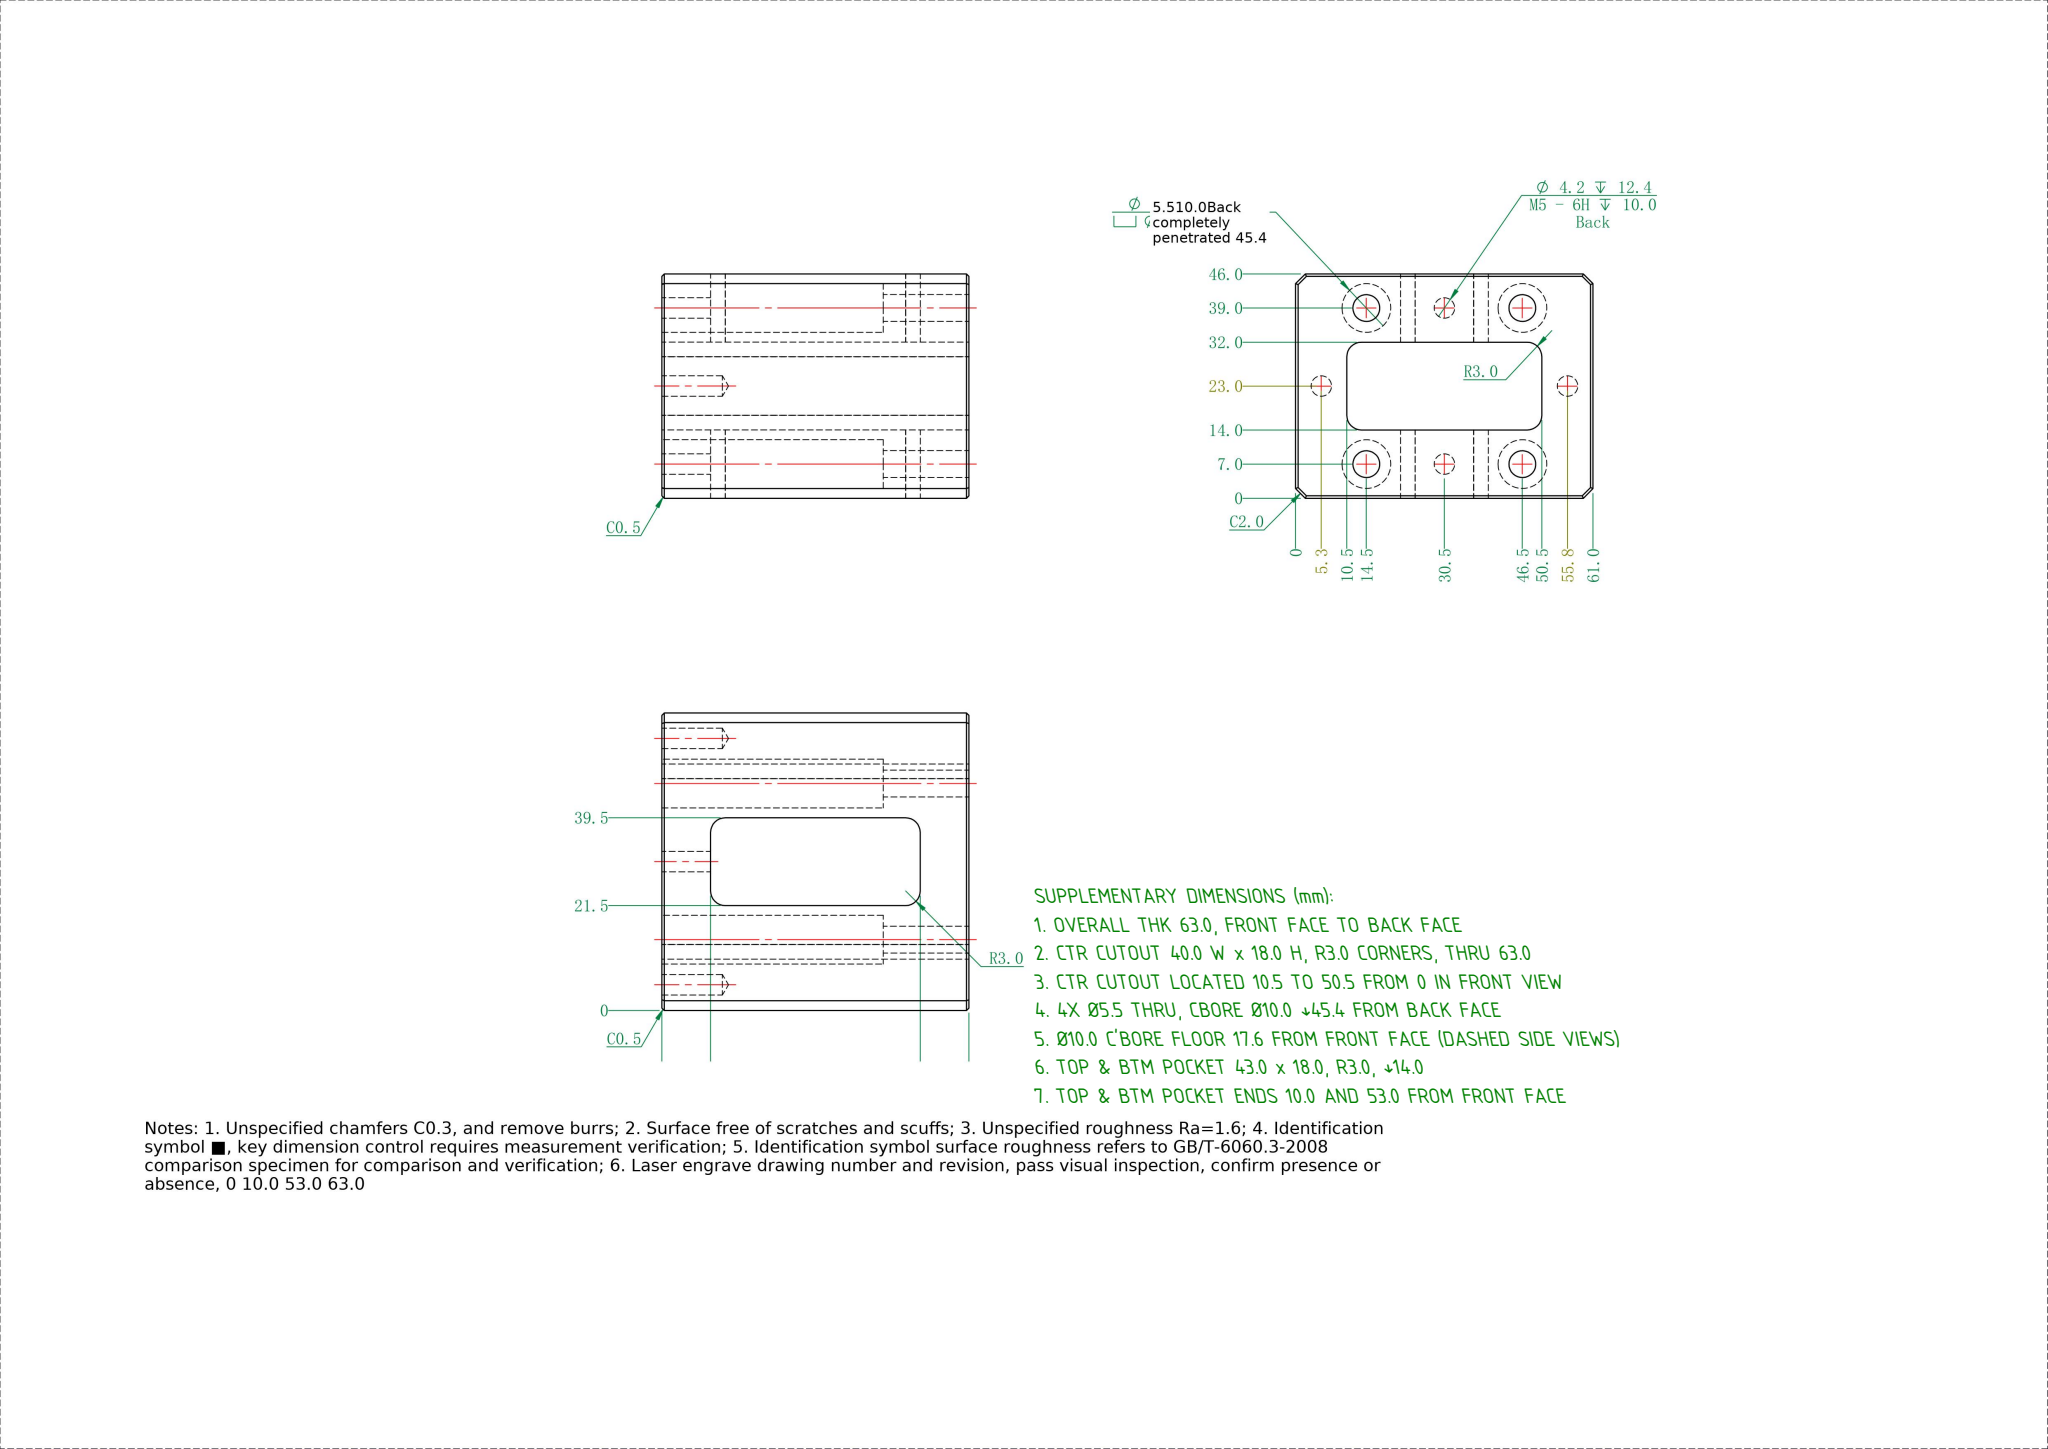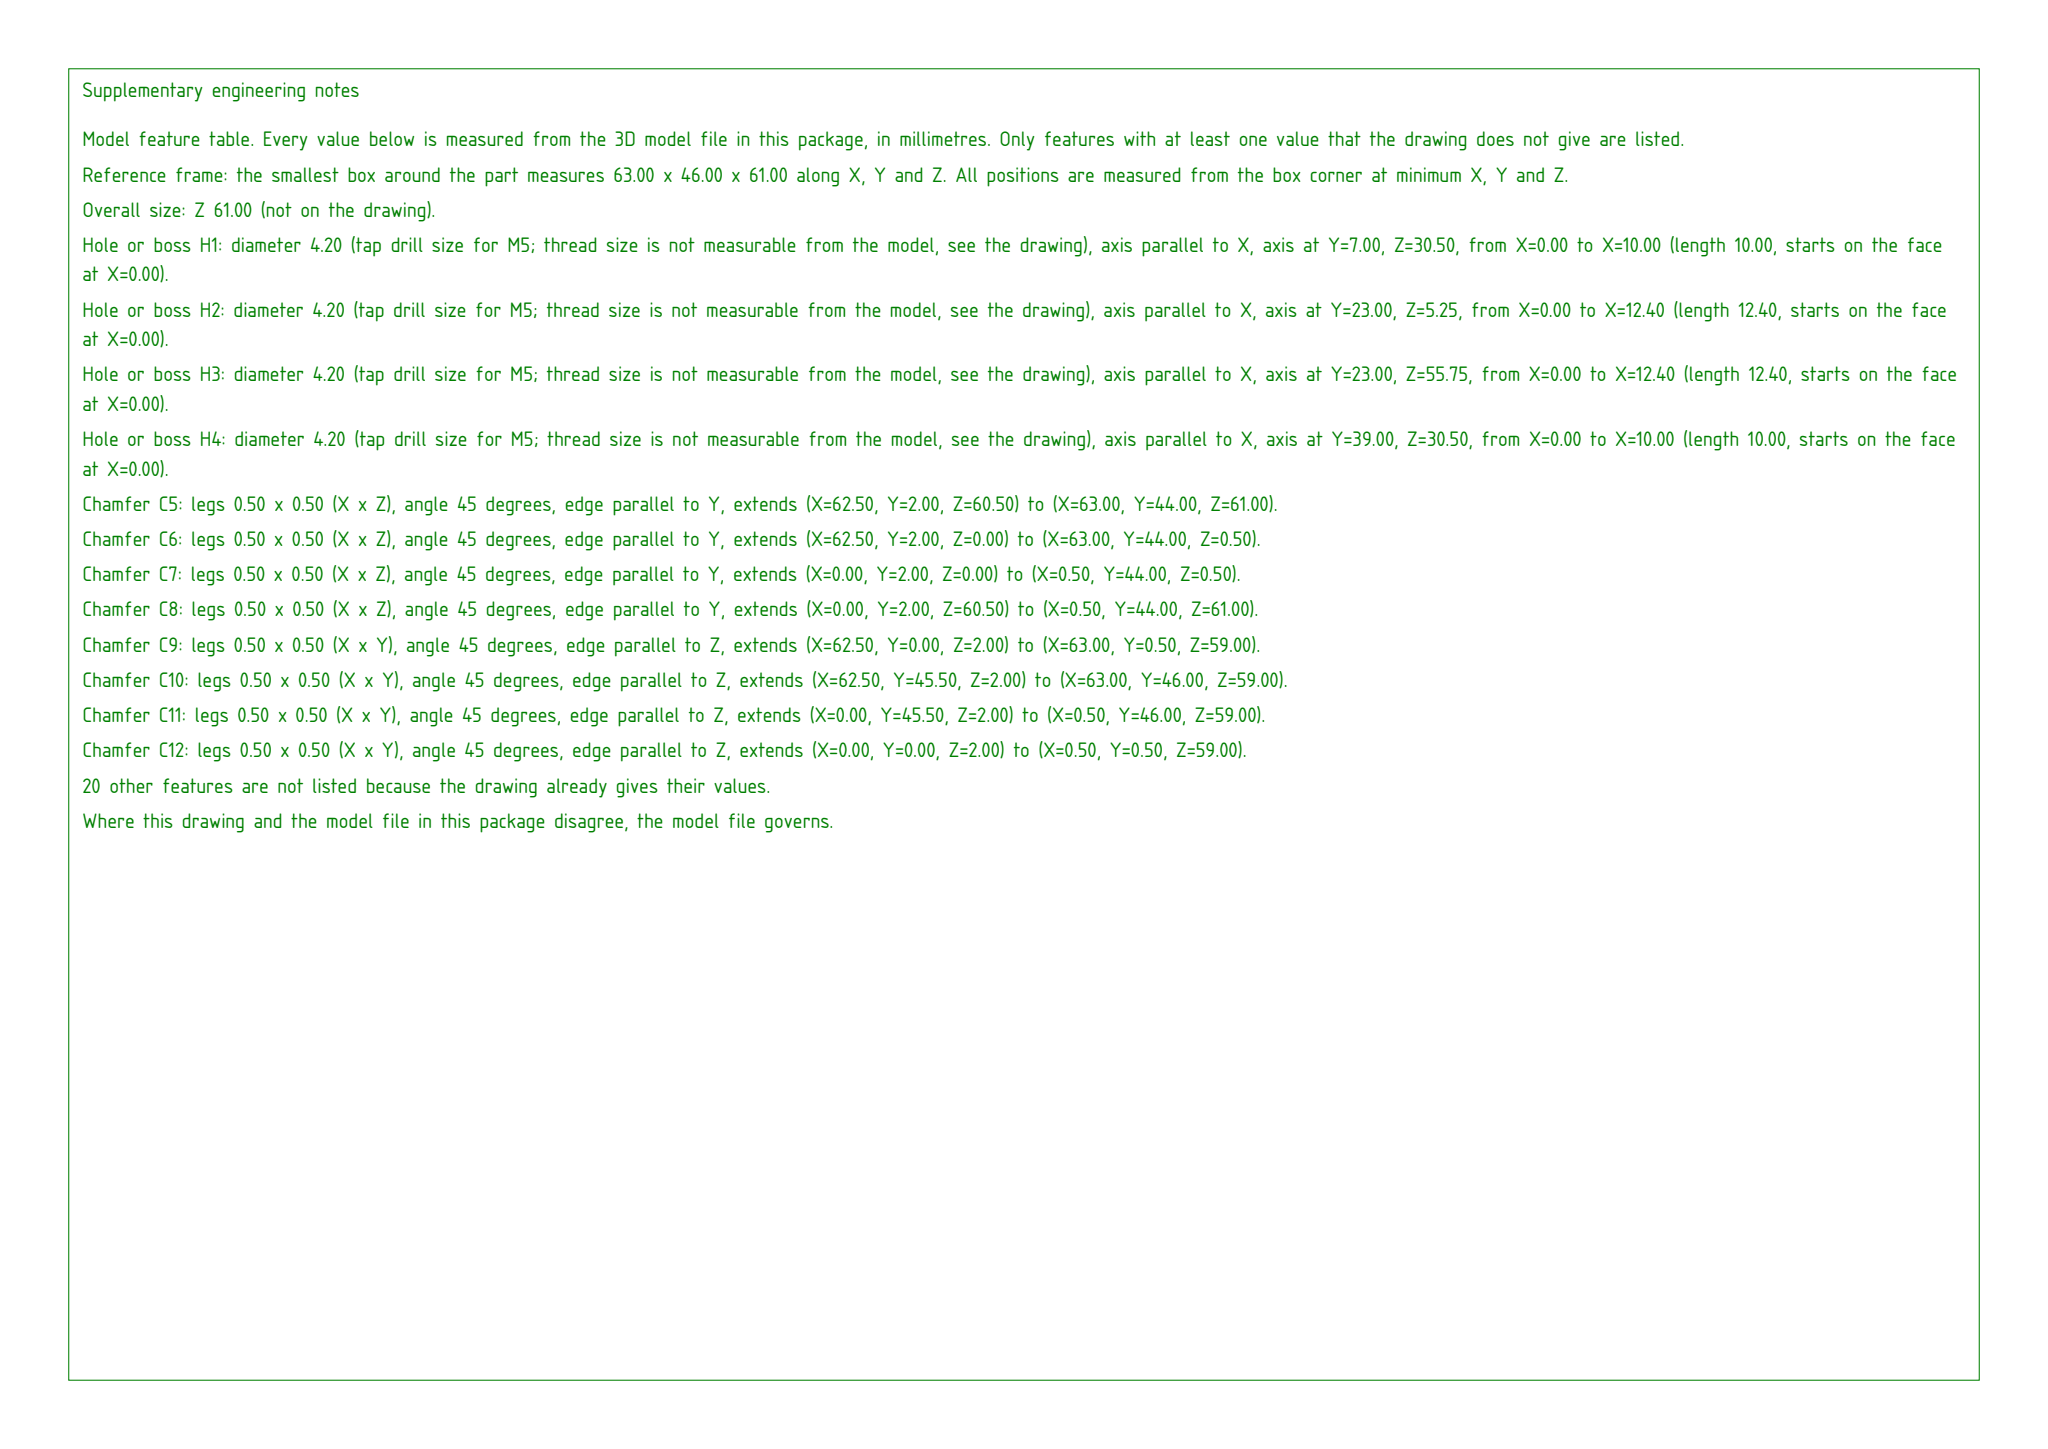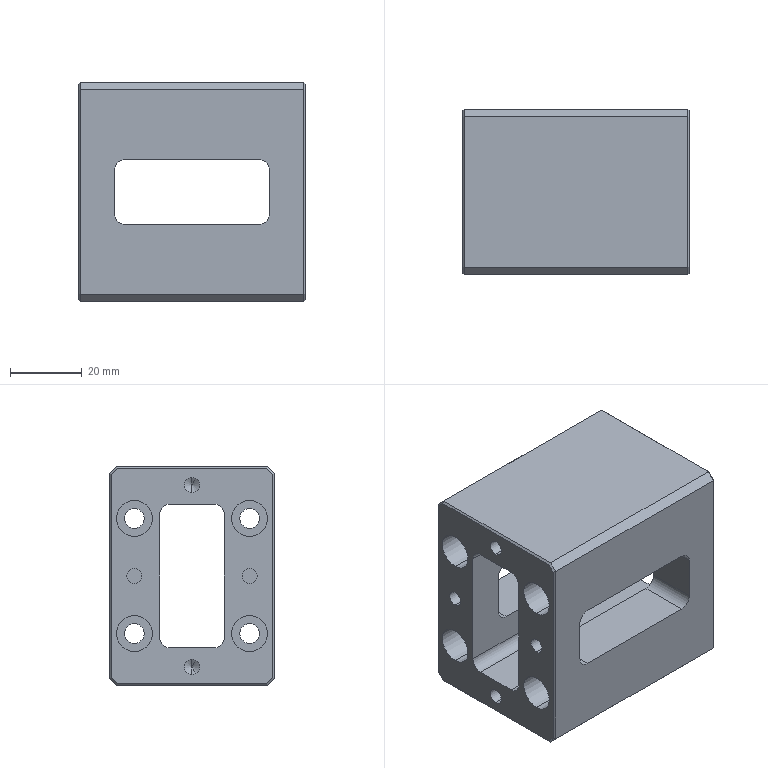Part | SolidWorks | mm | 1 solid | 82 faces | box 63 x 46 x 61 mm | volume 93325 mm3 | plane 42 | cylinder 36 | cone 4 | commonest cylinder face diameters 6 x12 4.2 x8 10 x8 5.5 x8
build123d program:
from build123d import *

# Parameters (mm, degrees)
SKETCH1_W                                       = 63
SKETCH1_H                                       = 46
BOSS_EXTRUDE1_DEPTH                             = 61
M5_HEX_SOCKET_HEAD_CAP_SCREW_CBORE1_D           = 5.5
M5_HEX_SOCKET_HEAD_CAP_SCREW_CBORE1_CBORE_D     = 10
M5_HEX_SOCKET_HEAD_CAP_SCREW_CBORE1_CBORE_DEPTH = 45.4
SKETCH4_W                                       = 40
SKETCH4_H                                       = 18
CUT_EXTRUDE1_DEPTH                              = 100.025
FILLET1_R                                       = 3
SKETCH5_W                                       = 43
SKETCH5_H                                       = 18
CUT_EXTRUDE2_DEPTH                              = 100.025
FILLET2_R                                       = 3
CHAMFER1_SIZE                                   = 2
M5_TAPPED_HOLE1_D                               = 4.2
M5_TAPPED_HOLE1_DEPTH                           = 12.4
M5_TAPPED_HOLE1_TIP                             = 1.262
CHAMFER2_SIZE                                   = 0.5


with BuildPart() as part:
    # Sketch1 → Boss-Extrude1 (new body)
    with BuildSketch(Plane.XY):
        with Locations((31.5, 23)):
            Rectangle(SKETCH1_W, SKETCH1_H)
    extrude(amount=BOSS_EXTRUDE1_DEPTH)

    # M5 Hex Socket Head Cap Screw CBORE1 (through all)
    with Locations(Plane.ZY):
        with Locations((46.5, 7), (14.5, 7), (14.5, 39), (46.5, 39)):
            CounterBoreHole(M5_HEX_SOCKET_HEAD_CAP_SCREW_CBORE1_D / 2, M5_HEX_SOCKET_HEAD_CAP_SCREW_CBORE1_CBORE_D / 2, M5_HEX_SOCKET_HEAD_CAP_SCREW_CBORE1_CBORE_DEPTH)

    # Sketch4 → Cut-Extrude1 (cut, through all)
    with BuildSketch(Plane.ZY):
        with Locations((30.5, 23)):
            Rectangle(SKETCH4_W, SKETCH4_H)
    extrude(amount=-CUT_EXTRUDE1_DEPTH, mode=Mode.SUBTRACT)

    # Fillet1
    fillet1_edges = [part.edges().sort_by_distance(p)[0] for p in [
        (31.5, 32, 50.5),
        (31.5, 14, 50.5),
        (31.5, 14, 10.5),
        (31.5, 32, 10.5),
    ]]
    fillet(fillet1_edges, radius=FILLET1_R)

    # Sketch5 → Cut-Extrude2 (cut, through all)
    with BuildSketch(Plane.XZ):
        with Locations((31.5, 30.5)):
            Rectangle(SKETCH5_W, SKETCH5_H)
    extrude(amount=-CUT_EXTRUDE2_DEPTH, mode=Mode.SUBTRACT)

    # Fillet2
    fillet2_edges = [part.edges().sort_by_distance(p)[0] for p in [
        (53, 7, 39.5),
        (53, 39, 39.5),
        (53, 7, 21.5),
        (53, 39, 21.5),
        (10, 7, 21.5),
        (10, 39, 21.5),
        (10, 7, 39.5),
        (10, 39, 39.5),
    ]]
    fillet(fillet2_edges, radius=FILLET2_R)

    # Chamfer1
    chamfer1_edges = [part.edges().sort_by_distance(p)[0] for p in [
        (31.5, 46, 61),
        (31.5, 46, 0),
        (31.5, 0, 0),
        (31.5, 0, 61),
    ]]
    chamfer(chamfer1_edges, length=CHAMFER1_SIZE)

    # M5 Tapped Hole1
    with Locations(Plane.ZY):
        with Locations((30.5, 39), (55.75, 23), (30.5, 7), (5.25, 23)):
            Hole(M5_TAPPED_HOLE1_D / 2, depth=M5_TAPPED_HOLE1_DEPTH)
            with Locations((0, 0, -(M5_TAPPED_HOLE1_DEPTH + M5_TAPPED_HOLE1_TIP / 2))):  # 118° drill point
                Cone(0, M5_TAPPED_HOLE1_D / 2, M5_TAPPED_HOLE1_TIP, mode=Mode.SUBTRACT)

    # Chamfer2
    chamfer2_edges = [part.edges().sort_by_distance(p)[0] for p in [
        (0, 23, 61),
        (63, 23, 61),
        (0, 23, 0),
        (0, 0, 30.5),
        (0, 46, 30.5),
        (0, 45, 1),
        (0, 1, 1),
        (0, 1, 60),
        (0, 45, 60),
        (63, 46, 30.5),
        (63, 23, 0),
        (63, 0, 30.5),
        (63, 45, 1),
        (63, 1, 1),
        (63, 1, 60),
        (63, 45, 60),
    ]]
    chamfer(chamfer2_edges, length=CHAMFER2_SIZE)


solid = part.part